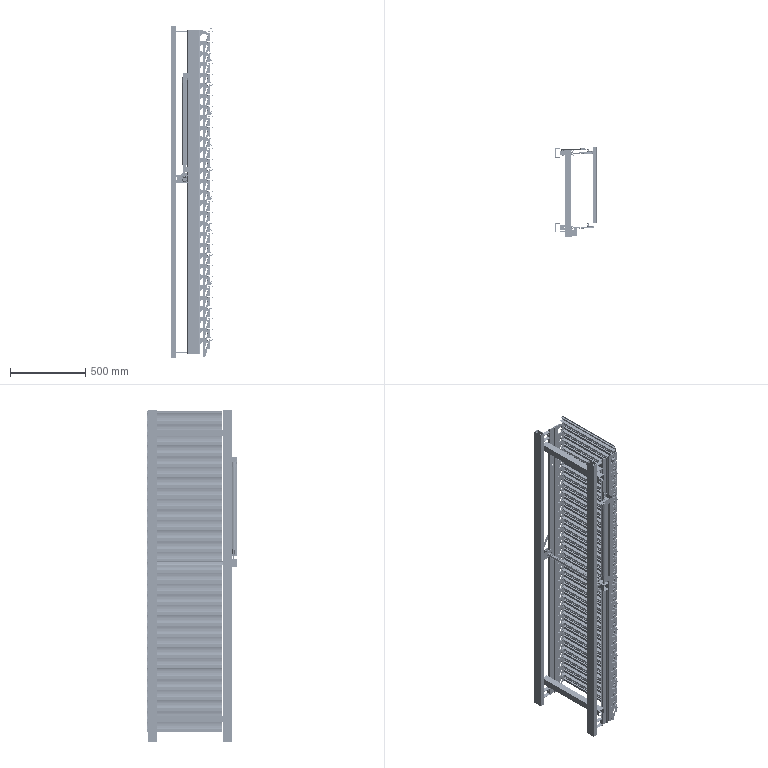Assembly | SolidWorks | mm | 178 component files | 361 solids | 14809 faces | box 272.21 x 596.66 x 2200 mm | volume 8172042 mm3 | plane 9210 | cylinder 4066 | torus 840 | spline 400 | cone 293 | commonest cylinder face diameters 2 x1398 7 x360 140 x360 15 x360 6 x252 10 x250 136 x180 10.189 x120
Bill of materials:
BeltDrive | 1 |  | Solid cylindrical shaft joined to a thin disc whose rim has a narrow band of axial teeth between two smooth side flanges; the disc has two off-center through holes.
Blade | 30 |  | Long, thin-walled, open extruded profile with a gently curved main wall, two inward flanges of different lengths, and a stepped C-shaped return at one edge.
Drive | 1 |  | Long hollow prism whose outer cross-section is an irregular hexagon, with a square bore running all the way through and four small rectangular fins sticking out on the outside.
DriveBar | 2 |  | Very long, slender strip with a U-shaped channel cross-section: a flat base and two upright side lips with rounded tops.
DriveBracketBase | 1 |  | Plate-type clip with two split cylindrical ring collars along one side and a perpendicular edge flange with two tapered (dovetail or barb-like) tabs on the other side.
DrivePart | 1 |  | Hub with a toothed flange: a cylindrical sleeve with a round bore and one keyway, joined to a larger disc that has a fine-toothed rim between side flanges and four through holes.
DriveShaft2 | 2 |  | Stepped shaft: a square-section bar section followed by a smaller round shaft section with a raised rectangular key with rounded ends near its free end.
Motor | 1 |  | Long, slender cylindrical body (faceted in the render) with a short cap at one end and stepped smaller-diameter shaft sections at the other end.
MotorCover | 1 |  | Long, thin angle profile (two legs meeting at a corner) with one long rectangular slot through one leg.
MotorDriveShaft | 1 |  | Short cylindrical base with a square prism post rising coaxially from one face.
MotorHeadBracket | 1 |  | L-shaped bent sheet bracket: a base plate with a stepped notch and a square hole, and an upright leg with two horizontal obround slots.
NormalGear | 2 |  | Straight-tooth bevel gear with a flat back face and a central bore that has keyway-like notches.
Part1^LouverMechanism2 | 1 |  | Slender flat bar of constant thickness. One end has an obround (stadium-shaped) pad set across the bar, joined with fillets; the other end is rounded.
ProtectiveCover | 1 |  | Thin-walled box shell, open on at least one face. A plate on top has a circular feature, and two parallel flat prongs stick out from one side to form a fork.
RackArm | 2 |  | Long straight extruded profile with a complex constant cross-section: a central web, a perpendicular flange with rounded ends partway along, a C-shaped channel with lips at one end, and a channel-like slotted feature with tapered lips at the other end.
ReversingArm | 60 |  | Curved flat lever-shaped plate. It has a boss with a through hole near the upper end, a slot at the top end, and a rounded paddle at the lower end. A cylindrical pin sticks out near the lower end, and a cylindrical post with a slotted head rises from one face.
ReversingArmBracket | 60 |  | Flat plate with a straight rectangular leg and a curved, tapering arm that sweeps out from the top of the leg. A large arch-shaped cutout lies between them, and a small cylindrical pin sticks out of the face at the rounded tip of the arm.
SquareAluminumTube | 2 |  | Long straight thin-walled rectangular channel. The bottom is open along its length, with a slot between two inward-turned stepped lips.
SquareIronTube | 2 |  | Long, slender, thin-walled rectangular hollow tube with an open rectangular section.
Stabilizer | 2 |  | Open-topped frame made of two parallel side walls joined by a cross wall. The lower edges of the side walls have semicircular cutouts of two sizes. A split end wall has stepped inner edges, and two small flat tabs with holes sit at the base of that end.
U-shapedFixingBracket | 4 |  | Bent strip bracket of constant thickness. It has a U-shaped central section and two outward flanges at the open ends. The flanges have rounded ends and holes, each leg of the U has a hole, and the closed end has a smaller hole.
Mates:
1. coincident | RackArm-2 face at (25.707, 6.747, 1891.064) dir (0, 1, 0) | ReversingArmBracket-1 face at (22.207, 6.747, 1820.664) dir (0, -1, 0)
2. coincident | RackArm-2 face at (22.207, 6.747, 1891.064) dir (1, 0, 0) | ReversingArmBracket-1 face at (22.207, 6.747, 1891.064) dir (-1, 0, 0)
3. coincident | ReversingArmBracket-1 face at (22.207, 6.747, 1820.664) dir (0, 0, -1) | ReversingArmBracket-60 face at (32.707, 6.747, 1820.664) dir (0, 0, 1)
4. coincident | RackArm-2 face at (22.207, 10.747, 1891.064) dir (0, -1, 0) | ReversingArmBracket-60 face at (22.207, 10.747, 1750.264) dir (0, 1, 0)
5. coincident | RackArm-2 face at (32.707, 10.747, 1891.064) dir (1, 0, 0) | ReversingArmBracket-60 face at (32.707, 5.747, 1820.664) dir (-1, 0, 0)
6. concentric | ReversingArmBracket-1 face at (96.249, 18.247, 1853.638) dir (0, -1, 0) r 3.5 | ReversingArm-1 edge at (96.249, 20.247, 1853.638) dir (0, 1, 0) r 3.5
7. parallel | RackArm-2 face at (32.707, 13.247, 1891.064) dir (0, 1, 0) | DriveBar-1 face at (57.241, 23.247, -367.352) dir (0, 1, 0)
8. coincident | ReversingArmBracket-1 face at (22.207, 12.247, 1820.664) dir (0, 1, 0) | ReversingArm-1 face at (96.249, 12.247, 1853.638) dir (0, -1, 0)
9. coincident | ReversingArmBracket-62 face at (22.207, 6.747, 1679.864) dir (0, 0, -1) | ReversingArmBracket-64 face at (32.707, 6.747, 1679.864) dir (0, 0, 1)
10. coincident | ReversingArmBracket-62 face at (36.207, 5.747, 1679.864) dir (1, 0, 0) | ReversingArmBracket-64 face at (36.207, 5.747, 1609.464) dir (1, 0, 0)
11. coincident | ReversingArmBracket-62 face at (22.207, 6.747, 1679.864) dir (0, -1, 0) | ReversingArmBracket-64 face at (22.207, 6.747, 1609.464) dir (0, -1, 0)
12. coincident | ReversingArmBracket-64 face at (22.207, 6.747, 1609.464) dir (0, -1, 0) | ReversingArmBracket-66 face at (22.207, 6.747, 1539.064) dir (0, -1, 0)
13. coincident | ReversingArmBracket-64 face at (22.207, 6.747, 1609.464) dir (0, 0, -1) | ReversingArmBracket-66 face at (32.707, 6.747, 1609.464) dir (0, 0, 1)
14. coincident | ReversingArmBracket-64 face at (22.207, 6.747, 1679.864) dir (-1, 0, 0) | ReversingArmBracket-66 face at (22.207, 6.747, 1609.464) dir (-1, 0, 0)
15. coincident | ReversingArmBracket-66 face at (22.207, 6.747, 1539.064) dir (0, 0, -1) | ReversingArmBracket-68 face at (32.707, 6.747, 1539.064) dir (0, 0, 1)
16. coincident | ReversingArmBracket-66 face at (22.207, 6.747, 1539.064) dir (0, -1, 0) | ReversingArmBracket-68 face at (22.207, 6.747, 1468.664) dir (0, -1, 0)
17. coincident | ReversingArmBracket-66 face at (22.207, 6.747, 1609.464) dir (-1, 0, 0) | ReversingArmBracket-68 face at (22.207, 6.747, 1539.064) dir (-1, 0, 0)
18. coincident | ReversingArmBracket-68 face at (22.207, 6.747, 1539.064) dir (-1, 0, 0) | ReversingArmBracket-70 face at (22.207, 6.747, 1468.664) dir (-1, 0, 0)
19. coincident | ReversingArmBracket-68 face at (22.207, 6.747, 1468.664) dir (0, 0, -1) | ReversingArmBracket-70 face at (32.707, 6.747, 1468.664) dir (0, 0, 1)
20. coincident | ReversingArmBracket-68 face at (22.207, 6.747, 1468.664) dir (0, -1, 0) | ReversingArmBracket-70 face at (22.207, 6.747, 1398.264) dir (0, -1, 0)
21. coincident | ReversingArmBracket-70 face at (22.207, 6.747, 1398.264) dir (0, -1, 0) | ReversingArmBracket-72 face at (22.207, 6.747, 1327.864) dir (0, -1, 0)
22. coincident | ReversingArmBracket-70 face at (22.207, 6.747, 1468.664) dir (-1, 0, 0) | ReversingArmBracket-72 face at (22.207, 6.747, 1398.264) dir (-1, 0, 0)
23. coincident | ReversingArmBracket-70 face at (22.207, 6.747, 1398.264) dir (0, 0, -1) | ReversingArmBracket-72 face at (32.707, 6.747, 1398.264) dir (0, 0, 1)
24. coincident | ReversingArmBracket-72 face at (22.207, 6.747, 1327.864) dir (0, 0, -1) | ReversingArmBracket-76 face at (32.707, 6.747, 1327.864) dir (0, 0, 1)
25. coincident | ReversingArmBracket-72 face at (22.207, 6.747, 1327.864) dir (0, -1, 0) | ReversingArmBracket-76 face at (22.207, 6.747, 1257.464) dir (0, -1, 0)
26. coincident | ReversingArmBracket-72 face at (36.207, 5.747, 1327.864) dir (1, 0, 0) | ReversingArmBracket-76 face at (36.207, 5.747, 1257.464) dir (1, 0, 0)
27. coincident | ReversingArmBracket-74 face at (36.207, 5.747, 1187.064) dir (1, 0, 0) | ReversingArmBracket-76 face at (36.207, 5.747, 1257.464) dir (1, 0, 0)
28. coincident | ReversingArmBracket-74 face at (22.207, 6.747, 1187.064) dir (0, -1, 0) | ReversingArmBracket-76 face at (22.207, 6.747, 1257.464) dir (0, -1, 0)
29. coincident | ReversingArmBracket-74 face at (32.707, 6.747, 1257.464) dir (0, 0, 1) | ReversingArmBracket-76 face at (22.207, 6.747, 1257.464) dir (0, 0, -1)
30. coincident | ReversingArmBracket-74 face at (22.207, 6.747, 1187.064) dir (0, 0, -1) | ReversingArmBracket-78 face at (32.707, 6.747, 1187.064) dir (0, 0, 1)
31. coincident | ReversingArmBracket-74 face at (22.207, 6.747, 1187.064) dir (0, -1, 0) | ReversingArmBracket-78 face at (22.207, 6.747, 1116.664) dir (0, -1, 0)
32. coincident | ReversingArmBracket-74 face at (36.207, 5.747, 1187.064) dir (1, 0, 0) | ReversingArmBracket-78 face at (36.207, 5.747, 1116.664) dir (1, 0, 0)
33. coincident | ReversingArmBracket-78 face at (36.207, 5.747, 1116.664) dir (1, 0, 0) | ReversingArmBracket-80 face at (36.207, 5.747, 1046.264) dir (1, 0, 0)
34. coincident | ReversingArmBracket-78 face at (22.207, 6.747, 1116.664) dir (0, -1, 0) | ReversingArmBracket-80 face at (22.207, 6.747, 1046.264) dir (0, -1, 0)
35. coincident | ReversingArmBracket-78 face at (22.207, 6.747, 1116.664) dir (0, 0, -1) | ReversingArmBracket-80 face at (32.707, 6.747, 1116.664) dir (0, 0, 1)
36. coincident | ReversingArmBracket-60 face at (22.207, 6.747, 1750.264) dir (0, 0, -1) | ReversingArmBracket-62 face at (32.707, 6.747, 1750.264) dir (0, 0, 1)
37. coincident | RackArm-2 face at (25.707, 6.747, 1891.064) dir (0, 1, 0) | ReversingArmBracket-62 face at (22.207, 6.747, 1679.864) dir (0, -1, 0)
38. coincident | ReversingArmBracket-60 face at (36.207, 5.747, 1750.264) dir (1, 0, 0) | ReversingArmBracket-62 face at (36.207, 5.747, 1679.864) dir (1, 0, 0)
39. coincident | ReversingArmBracket-82 face at (22.207, 6.747, 975.864) dir (0, 0, -1) | ReversingArmBracket-84 face at (32.707, 6.747, 975.864) dir (0, 0, 1)
40. coincident | ReversingArmBracket-82 face at (22.207, 6.747, 975.864) dir (0, -1, 0) | ReversingArmBracket-84 face at (22.207, 6.747, 905.464) dir (0, -1, 0)
41. coincident | ReversingArmBracket-82 face at (22.207, 6.747, 1046.264) dir (-1, 0, 0) | ReversingArmBracket-84 face at (22.207, 6.747, 975.864) dir (-1, 0, 0)
42. coincident | ReversingArmBracket-84 face at (22.207, 6.747, 905.464) dir (0, 0, -1) | ReversingArmBracket-86 face at (32.707, 6.747, 905.464) dir (0, 0, 1)
43. coincident | ReversingArmBracket-84 face at (36.207, 5.747, 905.464) dir (1, 0, 0) | ReversingArmBracket-86 face at (36.207, 5.747, 835.064) dir (1, 0, 0)
44. coincident | ReversingArmBracket-84 face at (22.207, 6.747, 905.464) dir (0, -1, 0) | ReversingArmBracket-86 face at (22.207, 6.747, 835.064) dir (0, -1, 0)
45. coincident | ReversingArmBracket-86 face at (22.207, 6.747, 835.064) dir (0, 0, -1) | ReversingArmBracket-88 face at (32.707, 6.747, 835.064) dir (0, 0, 1)
46. coincident | ReversingArmBracket-86 face at (22.207, 6.747, 835.064) dir (0, -1, 0) | ReversingArmBracket-88 face at (22.207, 6.747, 764.664) dir (0, -1, 0)
47. coincident | ReversingArmBracket-86 face at (36.207, 5.747, 835.064) dir (1, 0, 0) | ReversingArmBracket-88 face at (36.207, 5.747, 764.664) dir (1, 0, 0)
48. coincident | ReversingArmBracket-88 face at (22.207, 6.747, 764.664) dir (0, 0, -1) | ReversingArmBracket-92 face at (32.707, 6.747, 764.664) dir (0, 0, 1)
49. coincident | ReversingArmBracket-88 face at (22.207, 6.747, 764.664) dir (0, -1, 0) | ReversingArmBracket-92 face at (22.207, 6.747, 694.264) dir (0, -1, 0)
50. coincident | ReversingArmBracket-88 face at (36.207, 5.747, 764.664) dir (1, 0, 0) | ReversingArmBracket-92 face at (36.207, 5.747, 694.264) dir (1, 0, 0)
51. coincident | ReversingArmBracket-90 face at (36.207, 5.747, 623.864) dir (1, 0, 0) | ReversingArmBracket-92 face at (36.207, 5.747, 694.264) dir (1, 0, 0)
52. coincident | ReversingArmBracket-90 face at (22.207, 6.747, 623.864) dir (0, -1, 0) | ReversingArmBracket-92 face at (22.207, 6.747, 694.264) dir (0, -1, 0)
53. coincident | ReversingArmBracket-90 face at (32.707, 6.747, 694.264) dir (0, 0, 1) | ReversingArmBracket-92 face at (22.207, 6.747, 694.264) dir (0, 0, -1)
54. coincident | ReversingArmBracket-90 face at (22.207, 6.747, 623.864) dir (0, 0, -1) | ReversingArmBracket-94 face at (32.707, 6.747, 623.864) dir (0, 0, 1)
55. coincident | ReversingArmBracket-90 face at (22.207, 6.747, 623.864) dir (0, -1, 0) | ReversingArmBracket-94 face at (22.207, 6.747, 553.464) dir (0, -1, 0)
56. coincident | ReversingArmBracket-90 face at (36.207, 5.747, 623.864) dir (1, 0, 0) | ReversingArmBracket-94 face at (36.207, 5.747, 553.464) dir (1, 0, 0)
57. coincident | ReversingArmBracket-94 face at (22.207, 6.747, 553.464) dir (0, 0, -1) | ReversingArmBracket-96 face at (32.707, 6.747, 553.464) dir (0, 0, 1)
58. coincident | ReversingArmBracket-94 face at (36.207, 5.747, 553.464) dir (1, 0, 0) | ReversingArmBracket-96 face at (36.207, 5.747, 483.064) dir (1, 0, 0)
59. coincident | ReversingArmBracket-96 face at (22.207, 6.747, 483.064) dir (0, 0, -1) | ReversingArmBracket-98 face at (32.707, 6.747, 483.064) dir (0, 0, 1)
60. coincident | ReversingArmBracket-96 face at (36.207, 5.747, 483.064) dir (1, 0, 0) | ReversingArmBracket-98 face at (36.207, 5.747, 412.664) dir (1, 0, 0)
61. coincident | ReversingArmBracket-96 face at (22.207, 6.747, 483.064) dir (0, -1, 0) | ReversingArmBracket-98 face at (22.207, 6.747, 412.664) dir (0, -1, 0)
62. coincident | ReversingArmBracket-98 face at (22.207, 6.747, 412.664) dir (0, -1, 0) | ReversingArmBracket-100 face at (22.207, 6.747, 342.264) dir (0, -1, 0)
63. coincident | ReversingArmBracket-98 face at (22.207, 6.747, 412.664) dir (0, 0, -1) | ReversingArmBracket-100 face at (32.707, 6.747, 412.664) dir (0, 0, 1)
64. coincident | ReversingArmBracket-98 face at (36.207, 5.747, 412.664) dir (1, 0, 0) | ReversingArmBracket-100 edge at (36.207, 6.747, 412.664) dir (0, 1, 0)
65. coincident | ReversingArmBracket-100 face at (22.207, 6.747, 342.264) dir (0, 0, -1) | ReversingArmBracket-102 face at (32.707, 6.747, 342.264) dir (0, 0, 1)
66. coincident | ReversingArmBracket-100 face at (22.207, 6.747, 342.264) dir (0, -1, 0) | ReversingArmBracket-102 face at (22.207, 6.747, 271.864) dir (0, -1, 0)
67. coincident | ReversingArmBracket-100 face at (22.207, 6.747, 342.264) dir (0, -1, 0) | ReversingArmBracket-102 face at (22.207, 6.747, 271.864) dir (0, -1, 0)
68. coincident | ReversingArmBracket-100 face at (36.207, 5.747, 342.264) dir (1, 0, 0) | ReversingArmBracket-102 face at (36.207, 5.747, 271.864) dir (1, 0, 0)
69. coincident | ReversingArmBracket-80 face at (22.207, 6.747, 1046.264) dir (0, 0, -1) | ReversingArmBracket-82 face at (32.707, 6.747, 1046.264) dir (0, 0, 1)
70. coincident | RackArm-2 face at (25.707, 6.747, 1891.064) dir (0, 1, 0) | ReversingArmBracket-82 face at (22.207, 6.747, 975.864) dir (0, -1, 0)
71. coincident | ReversingArmBracket-80 face at (36.207, 5.747, 1046.264) dir (1, 0, 0) | ReversingArmBracket-82 face at (36.207, 5.747, 975.864) dir (1, 0, 0)
72. coincident | ReversingArmBracket-102 face at (22.207, 6.747, 271.864) dir (0, 0, -1) | ReversingArmBracket-104 face at (32.707, 6.747, 271.864) dir (0, 0, 1)
73. coincident | ReversingArmBracket-102 face at (22.207, 6.747, 271.864) dir (0, -1, 0) | ReversingArmBracket-104 face at (22.207, 6.747, 201.464) dir (0, -1, 0)
74. coincident | ReversingArmBracket-102 face at (36.207, 5.747, 271.864) dir (1, 0, 0) | ReversingArmBracket-104 face at (36.207, 5.747, 201.464) dir (1, 0, 0)
75. coincident | ReversingArmBracket-104 face at (22.207, 6.747, 201.464) dir (0, 0, -1) | ReversingArmBracket-106 face at (32.707, 6.747, 201.464) dir (0, 0, 1)
76. coincident | ReversingArmBracket-104 face at (22.207, 6.747, 201.464) dir (0, -1, 0) | ReversingArmBracket-106 face at (22.207, 6.747, 131.064) dir (0, -1, 0)
77. coincident | ReversingArmBracket-104 face at (36.207, 5.747, 201.464) dir (1, 0, 0) | ReversingArmBracket-106 face at (36.207, 5.747, 131.064) dir (1, 0, 0)
78. coincident | ReversingArmBracket-106 face at (36.207, 5.747, 131.064) dir (1, 0, 0) | ReversingArmBracket-108 face at (36.207, 5.747, 60.664) dir (1, 0, 0)
79. coincident | ReversingArmBracket-106 face at (22.207, 6.747, 131.064) dir (0, -1, 0) | ReversingArmBracket-108 face at (22.207, 6.747, 60.664) dir (0, -1, 0)
80. coincident | ReversingArmBracket-108 face at (36.207, 5.747, 60.664) dir (1, 0, 0) | ReversingArmBracket-110 face at (36.207, 5.747, -9.736) dir (1, 0, 0)
81. coincident | ReversingArmBracket-108 face at (22.207, 6.747, 60.664) dir (0, -1, 0) | ReversingArmBracket-110 face at (22.207, 6.747, -9.736) dir (0, -1, 0)
82. coincident | ReversingArmBracket-110 face at (36.207, 5.747, -9.736) dir (1, 0, 0) | ReversingArmBracket-112 face at (36.207, 5.747, -80.136) dir (1, 0, 0)
83. coincident | ReversingArmBracket-110 face at (22.207, 6.747, -9.736) dir (0, 0, -1) | ReversingArmBracket-112 face at (32.707, 6.747, -9.736) dir (0, 0, 1)
84. coincident | ReversingArmBracket-110 face at (22.207, 6.747, -9.736) dir (0, -1, 0) | ReversingArmBracket-112 face at (22.207, 6.747, -80.136) dir (0, -1, 0)
85. coincident | ReversingArmBracket-108 face at (22.207, 6.747, 60.664) dir (0, 0, -1) | ReversingArmBracket-110 face at (32.707, 6.747, 60.664) dir (0, 0, 1)
86. coincident | ReversingArmBracket-112 face at (22.207, 6.747, -80.136) dir (0, 0, -1) | ReversingArmBracket-114 face at (32.707, 6.747, -80.136) dir (0, 0, 1)
87. coincident | ReversingArmBracket-112 face at (22.207, 6.747, -80.136) dir (0, -1, 0) | ReversingArmBracket-114 face at (22.207, 6.747, -150.536) dir (0, -1, 0)
88. coincident | ReversingArmBracket-112 face at (36.207, 5.747, -80.136) dir (1, 0, 0) | ReversingArmBracket-114 face at (36.207, 5.747, -150.536) dir (1, 0, 0)
89. coincident | ReversingArmBracket-114 face at (36.207, 5.747, -150.536) dir (1, 0, 0) | ReversingArmBracket-116 face at (36.207, 5.747, -220.936) dir (1, 0, 0)
90. coincident | ReversingArmBracket-114 face at (22.207, 6.747, -150.536) dir (0, 0, -1) | ReversingArmBracket-116 face at (32.707, 6.747, -150.536) dir (0, 0, 1)
91. coincident | ReversingArmBracket-114 face at (22.207, 6.747, -150.536) dir (0, -1, 0) | ReversingArmBracket-116 face at (22.207, 6.747, -220.936) dir (0, -1, 0)
92. coincident | ReversingArmBracket-116 face at (22.207, 6.747, -220.936) dir (0, 0, -1) | assembly face at (32.707, -30.06, -220.936) dir (0, 0, 1)
93. coincident | ReversingArmBracket-116 face at (22.207, 6.747, -220.936) dir (0, -1, 0) | assembly face at (22.207, -30.06, -291.336) dir (0, -1, 0)
94. coincident | ReversingArmBracket-116 face at (36.207, 5.747, -220.936) dir (1, 0, 0) | assembly face at (36.207, -31.06, -291.336) dir (1, 0, 0)
95. coincident | ReversingArmBracket-94 face at (22.207, 6.747, 553.464) dir (0, 0, -1) | ReversingArmBracket-96 face at (32.707, 6.747, 553.464) dir (0, 0, 1)
96. coincident | ReversingArmBracket-94 face at (22.207, 6.747, 553.464) dir (0, -1, 0) | ReversingArmBracket-96 face at (22.207, 6.747, 483.064) dir (0, -1, 0)
97. concentric | DriveBar-1 face at (64.241, 73.247, 1631.848) dir (0, -1, 0) r 3.5 | ReversingArm-65 face at (64.241, 32.247, 1631.848) dir (0, -1, 0) r 3
98. coincident | ReversingArmBracket-62 edge at (96.249, 12.247, 1712.838) dir (0, 1, 0) r 3.5 | ReversingArm-65 edge at (96.249, 12.247, 1712.838) dir (0, -1, 0) r 3.5
99. coincident | ReversingArmBracket-60 face at (22.207, 12.247, 1750.264) dir (0, 1, 0) | ReversingArm-63 face at (96.249, 12.247, 1783.238) dir (0, -1, 0)
100. concentric | ReversingArmBracket-60 face at (96.249, 18.247, 1783.238) dir (0, -1, 0) r 3.5 | ReversingArm-63 face at (96.249, 20.247, 1783.238) dir (0, -1, 0) r 3.5
101. concentric | DriveBar-1 face at (64.241, 73.247, 1702.248) dir (0, -1, 0) r 3.5 | ReversingArm-63 face at (64.241, 32.247, 1702.248) dir (0, -1, 0) r 3
102. concentric | DriveBar-1 face at (64.241, 73.247, 1631.848) dir (0, -1, 0) r 3.5 | ReversingArm-65 face at (64.241, 32.247, 1631.848) dir (0, -1, 0) r 3
103. coincident | Motor-2 face at (-65.193, -32.853, 1552.064) dir (0, 0, 1) | MotorDriveShaft-1 face at (-65.193, -32.853, 1552.064) dir (0, 0, -1)
104. coincident | ReversingArm-1 face at (96.249, 20.247, 1853.638) dir (0, 1, 0) | DriveBar-1 face at (73.241, 20.247, -367.352) dir (0, -1, 0)
105. concentric | ReversingArm-1 face at (64.241, 32.247, 1772.648) dir (0, -1, 0) r 3 | DriveBar-1 face at (64.241, 73.247, 1772.648) dir (0, -1, 0) r 3.5
106. coincident | RackArm-3 face at (-45.793, 510.147, 1891.064) dir (-1, 0, 0) | SquareAluminumTube-2 face at (-45.793, 523.197, 1742.064) dir (1, 0, 0)
107. width | SquareAluminumTube-2 face at (-67.793, 523.197, 1764.064) dir (0, 1, 0) | SquareAluminumTube-2 face at (-67.793, -12.803, 1764.064) dir (0, -1, 0) | RackArm-3 face at (-36.793, 509.647, 1891.064) dir (0, 1, 0) | RackArm-2 face at (-43.793, 0.747, 1891.064) dir (0, -1, 0)
108. distance | SquareAluminumTube-2 face at (-45.793, 523.197, 1786.064) dir (0, 0, 1) | RackArm-2 face at (33.407, 5.247, 1891.064) dir (0, 0, 1)
109. width | SquareAluminumTube-3 face at (-67.793, -12.803, -131.936) dir (0, -1, 0) | SquareAluminumTube-3 face at (-67.793, 523.197, -131.936) dir (0, 1, 0) | RackArm-2 face at (-43.793, 0.747, 1891.064) dir (0, -1, 0) | RackArm-3 face at (-36.793, 509.647, 1891.064) dir (0, 1, 0)
110. coincident | RackArm-3 face at (-45.793, 499.247, 1891.064) dir (-1, 0, 0) | SquareAluminumTube-3 face at (-45.793, 523.197, -153.936) dir (1, 0, 0)
111. distance | RackArm-3 face at (33.407, 499.247, -258.936) dir (0, 0, -1) | SquareAluminumTube-3 face at (-45.793, 523.197, -153.936) dir (0, 0, -1)
112. coincident | Motor-2 face at (-65.193, -32.853, 1574.064) dir (0, 0, 1) | MotorHeadBracket-1 face at (-79.293, -47.753, 1574.064) dir (0, 0, -1)
113. coincident | MotorDriveShaft-1 face at (-70.193, -27.853, 1569.064) dir (0, 1, 0) | MotorHeadBracket-1 face at (-70.193, -27.853, 1577.064) dir (0, -1, 0)
114. coincident | MotorDriveShaft-1 face at (-70.193, -27.853, 1569.064) dir (-1, 0, 0) | MotorHeadBracket-1 face at (-70.193, -27.853, 1577.064) dir (1, 0, 0)
115. coincident | RackArm-2 face at (-36.793, 7.247, 1891.064) dir (0, -1, 0) | MotorCover-1 face at (-7.293, 7.247, 946.064) dir (0, 1, 0)
116. coincident | MotorCover-1 face at (-7.293, 6.747, 946.064) dir (-1, 0, 0) | MotorHeadBracket-1 face at (-7.293, -47.753, 1577.064) dir (1, 0, 0)
117. coincident | MotorCover-1 face at (-10.293, 6.747, 946.064) dir (0, -1, 0) | MotorHeadBracket-1 face at (-7.293, 6.747, 1577.064) dir (0, 1, 0)
118. parallel | RackArm-2 face at (-1.793, 7.247, 1891.064) dir (-1, 0, 0) | MotorHeadBracket-1 face at (-7.293, -47.753, 1577.064) dir (1, 0, 0)
119. distance | MotorCover-1 face at (-7.293, -54.253, 1606.064) dir (0, 0, 1) | MotorHeadBracket-1 face at (-79.293, -47.753, 1626.064) dir (0, 0, 1)
120. width | U-shapedFixingBracket-1 face at (-118.793, -4.303, 1881.064) dir (0, -1, 0) | U-shapedFixingBracket-1 face at (-118.793, 20.697, 1881.064) dir (0, 1, 0) | RackArm-2 face at (-36.793, 15.647, 1891.064) dir (0, 1, 0) | RackArm-2 face at (-43.793, 0.747, 1891.064) dir (0, -1, 0)
121. coincident | RackArm-2 face at (-45.793, 5.247, 1891.064) dir (-1, 0, 0) | U-shapedFixingBracket-1 face at (-45.793, -4.303, 1881.064) dir (1, 0, 0)
122. distance | U-shapedFixingBracket-1 face at (-118.793, -4.303, 1881.064) dir (0, 0, 1) | RackArm-2 face at (33.407, 5.247, 1891.064) dir (0, 0, 1)
123. width | U-shapedFixingBracket-2 face at (-118.793, 514.697, 1881.064) dir (0, 1, 0) | U-shapedFixingBracket-2 face at (-118.793, 489.697, 1881.064) dir (0, -1, 0) | RackArm-3 face at (-43.793, 494.747, 1891.064) dir (0, -1, 0) | RackArm-3 face at (-36.793, 509.647, 1891.064) dir (0, 1, 0)
124. coincident | RackArm-3 face at (-45.793, 510.147, 1891.064) dir (-1, 0, 0) | U-shapedFixingBracket-2 face at (-45.793, 489.697, 1881.064) dir (1, 0, 0)
125. coincident | U-shapedFixingBracket-1 face at (-118.793, -4.303, 1881.064) dir (0, 0, 1) | U-shapedFixingBracket-2 face at (-118.793, 489.697, 1881.064) dir (0, 0, 1)
126. coincident | Motor-2 face at (-65.193, -32.853, 946.564) dir (0, 0, -1) | assembly face at (-65.193, -32.853, 946.564) dir (0, 0, 1)
127. coincident | assembly face at (-90.193, -24.853, 910.564) dir (0, 1, 0) | assembly face at (-75.193, -24.853, 893.964) dir (0, -1, 0)
128. width | assembly face at (-75.193, -21.853, 893.964) dir (0, 0, -1) | assembly face at (-27.193, -21.853, 941.964) dir (0, 0, 1) | assembly face at (-68.193, -24.853, 898.564) dir (0, 0, -1) | assembly face at (-44.193, -24.853, 922.564) dir (0, 0, 1)
129. coincident | assembly face at (-44.193, -24.853, 898.564) dir (1, 0, 0) | assembly face at (-27.193, -83.853, 941.964) dir (-1, 0, 0)
130. coincident | Motor-2 face at (-61.36, -34.671, 927.064) dir (-0.3359, 0.9419, 0) | assembly face at (-68.193, -29.853, 956.564) dir (0, 1, 0)
131. coincident | Motor-2 face at (-67.011, -36.686, 927.064) dir (0.9419, 0.3359, 0) | assembly face at (-62.193, -29.853, 956.564) dir (1, 0, 0)
132. distance | MotorCover-1 face at (-6.793, -54.253, 946.064) dir (1, 0, 0) | RackArm-2 face at (-1.793, 7.247, 1891.064) dir (-1, 0, 0)
133. width | Drive-1 face at (-65.043, 25.197, 900.064) dir (0, -1, 0) | Drive-1 face at (-65.043, 485.197, 900.064) dir (0, 1, 0) | RackArm-2 face at (-36.793, 15.647, 1891.064) dir (0, 1, 0) | RackArm-3 face at (-43.793, 494.747, 1891.064) dir (0, -1, 0)
134. distance | MotorHeadBracket-1 face at (-79.293, -47.753, 1626.064) dir (0, 0, 1) | RackArm-2 face at (33.407, 5.247, 1891.064) dir (0, 0, 1)
135. concentric | assembly edge at (-65.193, -24.853, 910.564) dir (0, -1, 0) r 36 | assembly edge at (-65.193, -24.853, 910.564) dir (0, -1, 0) r 17.85
136. distance | U-shapedFixingBracket-3 face at (-45.793, 489.697, -248.936) dir (0, 0, -1) | RackArm-3 face at (33.407, 499.247, -258.936) dir (0, 0, -1)
137. coincident | RackArm-3 face at (-45.793, 510.147, 1891.064) dir (-1, 0, 0) | U-shapedFixingBracket-3 face at (-45.793, 489.697, -197.936) dir (1, 0, 0)
138. width | U-shapedFixingBracket-3 face at (-118.793, 514.697, -197.936) dir (0, 1, 0) | U-shapedFixingBracket-3 face at (-118.793, 489.697, -197.936) dir (0, -1, 0) | RackArm-3 face at (-36.793, 509.647, 1891.064) dir (0, 1, 0) | RackArm-3 face at (-43.793, 494.747, 1891.064) dir (0, -1, 0)
139. coincident | RackArm-2 face at (-45.793, 5.247, 1891.064) dir (-1, 0, 0) | U-shapedFixingBracket-4 face at (-45.793, -4.303, -197.936) dir (1, 0, 0)
140. distance | U-shapedFixingBracket-4 face at (-45.793, -4.303, -248.936) dir (0, 0, -1) | RackArm-2 face at (33.407, 5.247, -258.936) dir (0, 0, -1)
141. width | U-shapedFixingBracket-4 face at (-118.793, 20.697, -197.936) dir (0, 1, 0) | U-shapedFixingBracket-4 face at (-118.793, -4.303, -197.936) dir (0, -1, 0) | RackArm-2 face at (-43.793, 0.747, 1891.064) dir (0, -1, 0) | RackArm-2 face at (-36.793, 15.647, 1891.064) dir (0, 1, 0)
142. coincident | U-shapedFixingBracket-4 face at (-121.793, 20.697, -197.936) dir (-1, 0, 0) | SquareIronTube-1 face at (-121.793, 38.197, 1916.064) dir (1, 0, 0)
143. width | SquareIronTube-1 face at (-151.793, 38.197, -283.936) dir (0, 0, -1) | SquareIronTube-1 face at (-151.793, 38.197, 1916.064) dir (0, 0, 1) | U-shapedFixingBracket-4 face at (-121.793, -4.303, -275.936) dir (0, 0, -1) | U-shapedFixingBracket-1 face at (-121.793, -4.303, 1908.064) dir (0, 0, 1)
144. width | SquareIronTube-1 face at (-151.793, 38.197, 1916.064) dir (0, 1, 0) | SquareIronTube-1 face at (-121.793, -21.803, 1916.064) dir (0, -1, 0) | U-shapedFixingBracket-1 face at (-118.793, 20.697, 1881.064) dir (0, 1, 0) | U-shapedFixingBracket-1 face at (-118.793, -4.303, 1881.064) dir (0, -1, 0)
145. coincident | SquareIronTube-1 face at (-151.793, 38.197, 1916.064) dir (0, 0, 1) | SquareIronTube-2 face at (-151.793, 532.197, 1916.064) dir (0, 0, 1)
146. width | SquareIronTube-2 face at (-121.793, 472.197, 1916.064) dir (0, -1, 0) | SquareIronTube-2 face at (-151.793, 532.197, 1916.064) dir (0, 1, 0) | U-shapedFixingBracket-2 face at (-118.793, 489.697, 1881.064) dir (0, -1, 0) | U-shapedFixingBracket-2 face at (-118.793, 514.697, 1881.064) dir (0, 1, 0)
147. coincident | U-shapedFixingBracket-2 face at (-121.793, 514.697, 1881.064) dir (-1, 0, 0) | SquareIronTube-2 face at (-121.793, 532.197, 1916.064) dir (1, 0, 0)
148. coincident | assembly face at (-90.193, -24.853, 910.564) dir (0, 1, 0) | assembly face at (-65.193, -24.853, 910.564) dir (0, -1, 0)
149. parallel | RackArm-2 face at (-1.793, 9.247, 1891.064) dir (0, 1, 0) | assembly face at (-52.193, 27.247, 919.564) dir (0, -1, 0)
150. concentric | assembly edge at (-52.193, 51.347, 919.564) dir (0, -1, 0) r 18.45 | assembly edge at (-52.193, 32.247, 919.564) dir (0, 1, 0) r 3.5
151. width | assembly face at (-57.372, 32.247, 922.594) dir (-0.8631, 0, 0.505) | assembly face at (-47.015, 32.247, 916.533) dir (0.8631, 0, -0.505) | ReversingArm-80 face at (62.582, 33.247, 1065.009) dir (0.9716, 0, -0.2368) | ReversingArm-80 face at (64.04, 33.247, 1064.653) dir (-0.9716, 0, 0.2368)
152. coincident | ReversingArm-80 face at (64.241, 32.247, 1068.648) dir (0, -1, 0) | assembly face at (-52.193, 32.247, 919.564) dir (0, 1, 0)
153. concentric | DriveShaft2-2 face at (-65.043, 522.747, 900.064) dir (0, -1, 0) r 5 | assembly face at (-52.193, 526.247, 919.564) dir (0, -1, 0) r 3.5
154. coincident | ReversingArm-81 face at (64.241, 526.247, 1068.648) dir (0, -1, 0) | assembly face at (-52.193, 526.247, 919.564) dir (0, 1, 0)
155. concentric | ReversingArm-81 edge at (64.241, 526.247, 1068.648) dir (0, 1, 0) r 4 | assembly edge at (40.817, 526.247, 1082.116) dir (0, 1, 0) r 3.5
156. concentric | DriveShaft2-2 face at (-65.043, 522.747, 900.064) dir (0, -1, 0) r 5 | DrivePart-1 face at (-65.043, 521.247, 900.064) dir (0, -1, 0) r 7
157. concentric | DrivePart-1 face at (-69.412, 522.747, 915.456) dir (0, -1, 0) r 2.7 | assembly face at (-49.195, 521.197, 910.333) dir (0, 1, 0) r 2.7
158. coincident | DrivePart-1 face at (-65.043, 522.747, 900.064) dir (0, 1, 0) | assembly face at (-49.195, 521.197, 910.333) dir (0, -1, 0)
159. coincident | assembly face at (-49.193, 524.197, 910.564) dir (0, 1, 0) | assembly face at (-94.391, 524.197, 927.87) dir (0, -1, 0)
160. concentric | DrivePart-1 face at (-60.675, 522.747, 884.672) dir (0, -1, 0) r 2.7 | assembly face at (-61.23, 517.197, 895.062) dir (0, 1, 0) r 2.7
161. concentric | DrivePart-1 face at (-80.695, 521.197, 906.6) dir (0, -1, 0) r 2.7 | assembly face at (-80.695, 517.197, 906.6) dir (0, 1, 0) r 2.7
162. parallel | assembly face at (-49.193, 521.197, 915.564) dir (0, 0, 1) | assembly face at (-47.888, 527.197, 939.761) dir (-0.2477, 0, 0.9688)
163. concentric | ReversingArm-85 face at (64.241, 529.247, 927.848) dir (0, -1, 0) r 4 | assembly face at (28.775, 521.197, 910.333) dir (0, 1, 0) r 5
164. coincident | assembly face at (-49.193, 524.197, 910.564) dir (0, 1, 0) | assembly face at (-99.402, 524.197, 949.479) dir (0, -1, 0)
165. parallel | RackArm-3 face at (-43.793, 509.647, 1891.064) dir (1, 0, 0) | assembly face at (-51.402, 527.197, 901.479) dir (1, 0, 0)
166. slot | assembly face at (-75.402, 517.197, 909.479) dir (0, 1, 0) r 2.7 | assembly face at (-49.193, 521.197, 910.564) dir (0, 1, 0) r 2.7
167. coincident | RackArm-3 face at (-45.793, 510.147, 1891.064) dir (-1, 0, 0) | assembly face at (-45.793, 498.197, 950.979) dir (1, 0, 0)
168. coincident | assembly face at (-49.195, 524.197, 910.333) dir (0, 1, 0) | assembly face at (-98.32, 524.197, 836.032) dir (0, -1, 0)
169. coincident | RackArm-3 face at (-45.793, 510.147, 1891.064) dir (-1, 0, 0) | assembly face at (-45.793, 498.197, 1061.284) dir (1, 0, 0)
170. parallel | U-shapedFixingBracket-3 face at (-45.793, 489.697, -248.936) dir (0, 0, -1) | assembly face at (-49.195, 521.197, 905.333) dir (0, 0, -1)
171. parallel | SquareAluminumTube-2 face at (-45.793, 523.197, 1786.064) dir (0, 0, 1) | assembly face at (-17.802, 524.197, 930.775) dir (0, 0, 1)
172. concentric | ReversingArm-85 face at (64.241, 526.247, 927.848) dir (0, -1, 0) r 3 | assembly edge at (60.168, 527.197, 925.775) dir (0, 1, 0) r 3
173. coincident | RackArm-3 face at (-45.793, 510.147, 1891.064) dir (-1, 0, 0) | assembly face at (-45.793, 498.197, 884.003) dir (1, 0, 0)
174. coincident | assembly face at (-17.802, 527.197, 925.775) dir (0, 1, 0) | assembly face at (-89.193, 524.197, 933.503) dir (0, -1, 0)
175. coincident | DrivePart-1 face at (-65.043, 522.747, 900.064) dir (0, 1, 0) | assembly face at (-80.985, 520.247, 901.428) dir (0, -1, 0)
176. concentric | DrivePart-1 face at (-60.675, 522.747, 884.672) dir (0, -1, 0) r 2.7 | assembly face at (-49.102, 523.247, 898.699) dir (0, -1, 0) r 2.7
177. concentric | DrivePart-1 face at (-69.412, 522.747, 915.456) dir (0, -1, 0) r 2.7 | assembly face at (-80.985, 523.247, 901.428) dir (0, -1, 0) r 2.7
178. width | RackArm-3 face at (-1.793, 503.247, 1891.064) dir (0, 1, 0) | RackArm-3 face at (-36.793, 501.247, 1891.064) dir (0, -1, 0) | Stabilizer-1 face at (-36.793, 505.247, 927.064) dir (0, -1, 0) | Stabilizer-1 face at (-33.793, 499.247, 927.064) dir (0, 1, 0)
179. coincident | RackArm-3 face at (-36.793, 503.247, 1891.064) dir (1, 0, 0) | Stabilizer-1 face at (-36.793, 505.247, 927.064) dir (-1, 0, 0)
180. coincident | Stabilizer-1 face at (-33.793, 505.247, 927.064) dir (1, 0, 0) | Stabilizer-2 face at (-33.793, 516.247, 873.064) dir (1, 0, 0)
181. coincident | Stabilizer-1 face at (-33.793, 516.247, 927.064) dir (0, 1, 0) | Stabilizer-2 face at (-78.793, 516.247, 873.064) dir (0, 1, 0)
182. coincident | Stabilizer-1 face at (-78.793, 516.247, 900.064) dir (0, 0, -1) | Stabilizer-2 face at (-78.793, 488.247, 900.064) dir (0, 0, 1)
183. concentric | Motor-2 face at (-65.193, -32.853, 927.064) dir (0, 0, 1) r 5 | NormalGear-1 face at (-65.193, -32.853, 914.683) dir (0, 0, -1) r 5.008
184. coincident | RackArm-2 face at (-45.793, 5.247, 1891.064) dir (-1, 0, 0) | DriveBracketBase-1 face at (-45.793, 11.147, 946.064) dir (1, 0, 0)
185. coincident | RackArm-2 face at (-45.793, 11.147, 1891.064) dir (0, -1, 0) | DriveBracketBase-1 face at (-46.793, 11.147, 886.064) dir (0, 1, 0)
186. coincident | Motor-2 face at (-65.193, -32.853, 913.064) dir (0, 0, -1) | NormalGear-1 face at (-75.908, -34.78, 913.064) dir (0, 0, -1)
187. coincident | Drive-1 face at (-71.219, 25.197, 903.509) dir (0.273, 0, -0.962) | DriveShaft2-1 face at (-71.219, 65.197, 903.509) dir (-0.273, 0, 0.962)
188. coincident | Drive-1 face at (-71.219, 25.197, 903.509) dir (0.962, 0, 0.273) | DriveShaft2-1 face at (-68.488, 65.197, 893.889) dir (-0.962, 0, -0.273)
189. coincident | Drive-1 face at (-65.043, 25.197, 900.064) dir (0, -1, 0) | DriveShaft2-1 face at (-65.043, 25.197, 900.064) dir (0, -1, 0)
190. concentric | DriveBracketBase-1 face at (-65.043, 5.147, 900.064) dir (0, 1, 0) r 5 | DriveShaft2-1 face at (-65.043, -20.803, 900.064) dir (0, 1, 0) r 5
191. coincident | DriveShaft2-1 face at (-65.043, -20.803, 900.064) dir (0, -1, 0) | NormalGear-2 face at (-55.811, -20.803, 894.295) dir (0, -1, 0)
192. concentric | DriveShaft2-1 face at (-65.043, -20.803, 900.064) dir (0, 1, 0) r 5 | NormalGear-2 face at (-65.043, -19.183, 900.064) dir (0, -1, 0) r 5.008
193. coincident | Drive-1 face at (-71.219, 25.197, 903.509) dir (0.273, 0, -0.962) | DriveShaft2-2 face at (-71.219, 436.747, 903.509) dir (-0.273, 0, 0.962)
194. coincident | Drive-1 face at (-71.219, 25.197, 903.509) dir (0.962, 0, 0.273) | DriveShaft2-2 face at (-68.488, 436.747, 893.889) dir (-0.962, 0, -0.273)
195. coincident | DriveShaft2-2 face at (-65.043, 522.747, 900.064) dir (0, 1, 0) | DrivePart-1 face at (-65.043, 522.747, 900.064) dir (0, 1, 0)
196. concentric | DrivePart-1 face at (-65.043, 521.247, 900.064) dir (0, -1, 0) r 12 | Stabilizer-1 face at (-65.043, 479.247, 900.064) dir (0, 1, 0) r 12
197. gear | NormalGear-1 edge at (-65.193, -32.853, 923.08) dir (0, 0, -1) r 15.012 | NormalGear-2 edge at (-65.043, -10.787, 900.064) dir (0, -1, 0) r 15.012
198. coincident | DrivePart-1 face at (-65.043, 522.747, 900.064) dir (0, 1, 0) | assembly face at (-76.874, 520.247, 898.053) dir (0, -1, 0)
199. concentric | DrivePart-1 face at (-60.675, 522.747, 884.672) dir (0, -1, 0) r 2.7 | assembly face at (-53.213, 523.247, 902.075) dir (0, -1, 0) r 2.7
200. concentric | DrivePart-1 face at (-69.412, 522.747, 915.456) dir (0, -1, 0) r 2.7 | assembly face at (-76.874, 523.247, 898.053) dir (0, -1, 0) r 2.7
201. parallel | DriveShaft2-2 face at (-66.552, 521.747, 901.715) dir (-0.273, 0, 0.962) | DrivePart-1 face at (-59.436, 521.247, 904.254) dir (0.273, 0, -0.962)
202. coincident | DrivePart-1 face at (-65.043, 488.247, 900.064) dir (0, -1, 0) | Stabilizer-1 face at (-78.793, 488.247, 927.064) dir (0, -1, 0)
203. concentric | Stabilizer-2 face at (-102.554, 521.247, 900.064) dir (0, -1, 0) r 6.4 | BeltDrive-1 face at (-102.554, 484.247, 900.064) dir (0, 1, 0) r 5.4
204. coincident | Stabilizer-2 face at (-78.793, 516.247, 873.064) dir (0, 1, 0) | BeltDrive-1 face at (-102.554, 516.247, 900.064) dir (0, -1, 0)
205. coincident | SquareIronTube-1 face at (-121.793, 38.197, 1916.064) dir (1, 0, 0) | ProtectiveCover-1 face at (-121.793, -16.839, 2.984) dir (-1, 0, 0)
206. parallel | Motor-2 face at (-65.193, -32.853, 927.064) dir (0, 0, 1) r 5 | ProtectiveCover-1 face at (-64.669, -31.405, 891.714) dir (0, 0, 1) r 10.624
207. coincident | SquareIronTube-1 face at (-121.793, -21.803, 1916.064) dir (0, -1, 0) | ProtectiveCover-1 face at (-121.793, -21.803, 893.806) dir (0, -1, 0)
208. distance | ProtectiveCover-1 face at (-42.793, -54.859, 926.064) dir (0, 0, 1) | MotorCover-1 face at (-7.293, -54.253, 946.064) dir (0, 0, -1)
209. parallel | Blade-1 face at (101.142, 541.806, 1822.313) dir (-0.9999, 0, 0.0159) | ReversingArm-62 face at (101.248, 514.247, 1853.558) dir (0.9999, 0, -0.0159)
210. lock | Blade-1 reference at (0, 0, 0) dir (1, 0, 0) | ReversingArm-62 reference at (0, 0, 0) dir (1, 0, 0)
211. distance | Blade-17 face at (104.956, 541.806, 772.262) dir (-0.9999, 0, 0.0159) | Blade-16 face at (102.441, 541.806, 778.794) dir (0.9999, 0, -0.0159)
212. concentric | ReversingArm-119 face at (96.249, 514.247, -187.962) dir (0, -1, 0) r 3.5 | ReversingArmBracket-117 face at (96.249, 512.247, -187.962) dir (0, -1, 0) r 3.5
213. coincident | RackArm-3 face at (33.407, 499.247, 1891.064) dir (0, 0, 1) | ReversingArmBracket-59 face at (32.707, 500.747, 1891.064) dir (0, 0, 1)
214. concentric | BeltDrive-1 face at (-107.713, 517.747, 892.689) dir (0, -1, 0) r 2.5 | Part1^LouverMechanism2-1 face at (-107.713, 532.247, 892.689) dir (0, -1, 0) r 3.616
215. coincident | BeltDrive-1 face at (-102.554, 522.247, 900.064) dir (0, 1, 0) | Part1^LouverMechanism2-1 face at (40.321, 522.247, 1085.43) dir (0, -1, 0)
216. concentric | Motor-2 face at (-65.193, -32.853, 993.064) dir (0, 0, 1) r 17.5 | MotorDriveShaft-1 face at (-65.193, -32.853, 1567.064) dir (0, 0, 1) r 10